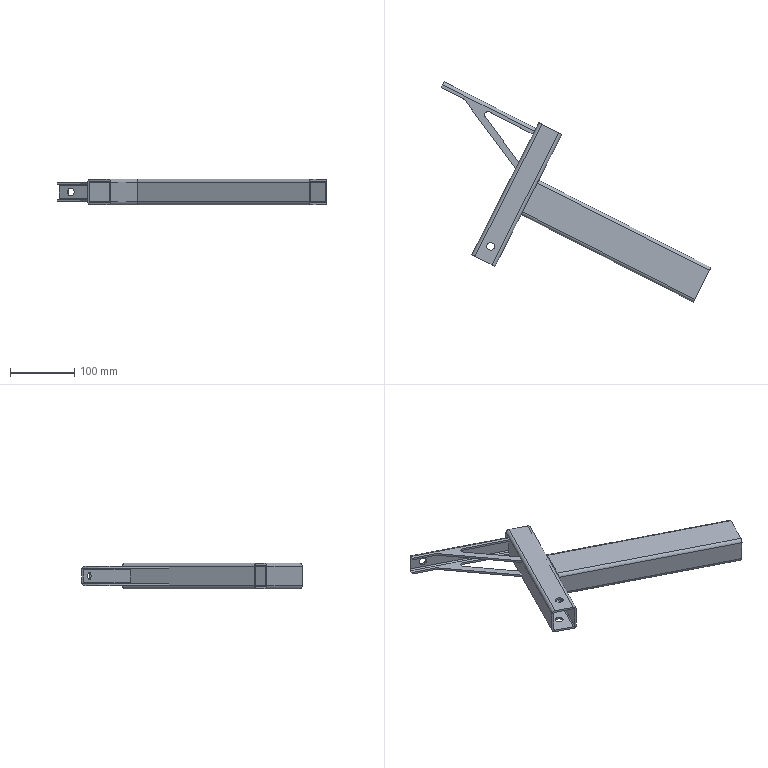Component | SolidWorks | FilmPressingSoilCoveringMechanism2Reverse-2_FilmPressingSoilWheelBracket-1 | 1 solid | 69 faces | box 418.86 x 342.01 x 40 mm | volume 288161 mm3 | plane 39 | cylinder 30 | commonest cylinder face diameters 10 x14 4 x10 12 x6
build123d program:
from build123d import *

# Parameters (mm, degrees)
BOSS_EXTRUDE1_DEPTH      = 150
BOSS_EXTRUDE2_DEPTH      = 80
BOSS_EXTRUDE2_DEPTH_BACK = 150
EXTRUDE_THIN1_DEPTH      = 160
BOSS_EXTRUDE3_DEPTH      = 3
FILLET1_R                = 5
SKETCH5_R                = 6
CUT_EXTRUDE1_DEPTH       = 373.156
SKETCH6_R                = 6
CUT_EXTRUDE2_DEPTH       = 300


with BuildPart() as part:
    # Sketch1 → Boss-Extrude1 (new, symmetric)
    with BuildSketch(Plane.XY):
        with BuildLine():
            Line((-15, -30), (15, -30))
            ThreePointArc((15, -30), (18.536, -28.536), (20, -25))
            Line((20, -25), (20, 25))
            ThreePointArc((20, 25), (18.536, 28.536), (15, 30))
            Line((15, 30), (-15, 30))
            ThreePointArc((-15, 30), (-18.536, 28.536), (-20, 25))
            Line((-20, 25), (-20, -25))
            ThreePointArc((-20, -25), (-18.536, -28.536), (-15, -30))
        make_face()
        with BuildLine():
            Line((-15, 27), (15, 27))
            ThreePointArc((15, 27), (16.414, 26.414), (17, 25))
            Line((17, 25), (17, -25))
            ThreePointArc((17, -25), (16.414, -26.414), (15, -27))
            Line((15, -27), (-15, -27))
            ThreePointArc((-15, -27), (-16.414, -26.414), (-17, -25))
            Line((-17, -25), (-17, 25))
            ThreePointArc((-17, 25), (-16.414, 26.414), (-15, 27))
        make_face(mode=Mode.SUBTRACT)
    extrude(amount=BOSS_EXTRUDE1_DEPTH, both=True)

    # Sketch2 → Boss-Extrude2 (add, two sides: drawn at the far end of the back side and taken through both)
    with BuildSketch(Plane(origin=(0, 30, 0), x_dir=(1, 0, 0), z_dir=(0, 1, 0)).offset(-BOSS_EXTRUDE2_DEPTH_BACK)):
        with BuildLine():
            Line((-15, 150), (15, 150))
            ThreePointArc((15, 150), (18.536, 151.464), (20, 155))
            Line((20, 155), (20, 185))
            ThreePointArc((20, 185), (18.536, 188.536), (15, 190))
            Line((15, 190), (-15, 190))
            ThreePointArc((-15, 190), (-18.536, 188.536), (-20, 185))
            Line((-20, 185), (-20, 155))
            ThreePointArc((-20, 155), (-18.536, 151.464), (-15, 150))
        make_face()
        with BuildLine():
            Line((-15, 187), (15, 187))
            ThreePointArc((15, 187), (16.414, 186.414), (17, 185))
            Line((17, 185), (17, 155))
            ThreePointArc((17, 155), (16.414, 153.586), (15, 153))
            Line((15, 153), (-15, 153))
            ThreePointArc((-15, 153), (-16.414, 153.586), (-17, 155))
            Line((-17, 155), (-17, 185))
            ThreePointArc((-17, 185), (-16.414, 186.414), (-15, 187))
        make_face(mode=Mode.SUBTRACT)
    extrude(amount=BOSS_EXTRUDE2_DEPTH + BOSS_EXTRUDE2_DEPTH_BACK)

    # Sketch3 → Extrude-Thin1 (add)
    with BuildSketch(Plane(origin=(0, 0, -190), x_dir=(-1, 0, 0), z_dir=(0, 0, -1))):
        with BuildLine():
            Line((-15, 90), (-15, 95))
            ThreePointArc((-15, 95), (-13.536, 98.536), (-10, 100))
            Line((-10, 100), (10, 100))
            ThreePointArc((10, 100), (13.536, 98.536), (15, 95))
            Line((15, 95), (15, 90))
            Line((15, 90), (12, 90))
            Line((12, 90), (12, 95))
            ThreePointArc((12, 95), (11.414, 96.414), (10, 97))
            Line((10, 97), (-10, 97))
            ThreePointArc((-10, 97), (-11.414, 96.414), (-12, 95))
            Line((-12, 95), (-12, 90))
            Line((-12, 90), (-15, 90))
        make_face()
    extrude(amount=EXTRUDE_THIN1_DEPTH)

    # Sketch4 → Boss-Extrude3 (add)
    with BuildSketch(Plane(origin=(15, 0, 0), x_dir=(0, 0, -1), z_dir=(1, 0, 0))):
        Polygon((190, 30), (310, 90), (287.639, 90), (190, 41.18), align=None)
    boss_extrude3 = extrude(amount=-BOSS_EXTRUDE3_DEPTH)

    # Mirror1: Boss-Extrude3 across plane
    add(boss_extrude3.mirror(Plane(origin=(0, 0, 0), x_dir=(0, 0, 1), z_dir=(1, 0, 0))))

    # Fillet1
    fillet1_edges = [part.edges().sort_by_distance(p)[0] for p in [
        (13.5, 90, -287.639),
        (13.5, 90, -310),
        (-13.5, 90, -310),
        (-13.5, 90, -287.639),
    ]]
    fillet(fillet1_edges, radius=FILLET1_R)

    # Sketch5 → Cut-Extrude1 (cut, through all)
    with BuildSketch(Plane(origin=(20, 0, 0), x_dir=(0, 0, -1), z_dir=(1, 0, 0))):
        with Locations((170, -95)):
            Circle(SKETCH5_R)
    extrude(amount=-CUT_EXTRUDE1_DEPTH, mode=Mode.SUBTRACT)

    # Sketch6 → Cut-Extrude2 (cut)
    with BuildSketch(Plane(origin=(0, 100, 0), x_dir=(1, 0, 0), z_dir=(0, 1, 0))):
        with Locations(Location((0, 330, 0), (0, 0, 270))):
            Circle(SKETCH6_R)
    extrude(amount=-CUT_EXTRUDE2_DEPTH, mode=Mode.SUBTRACT)


solid = part.part

# Placed as in the assembly
solid = solid.moved(Location((-1449.681, -353.984, 2567.971), (90, 63.121, -90)))